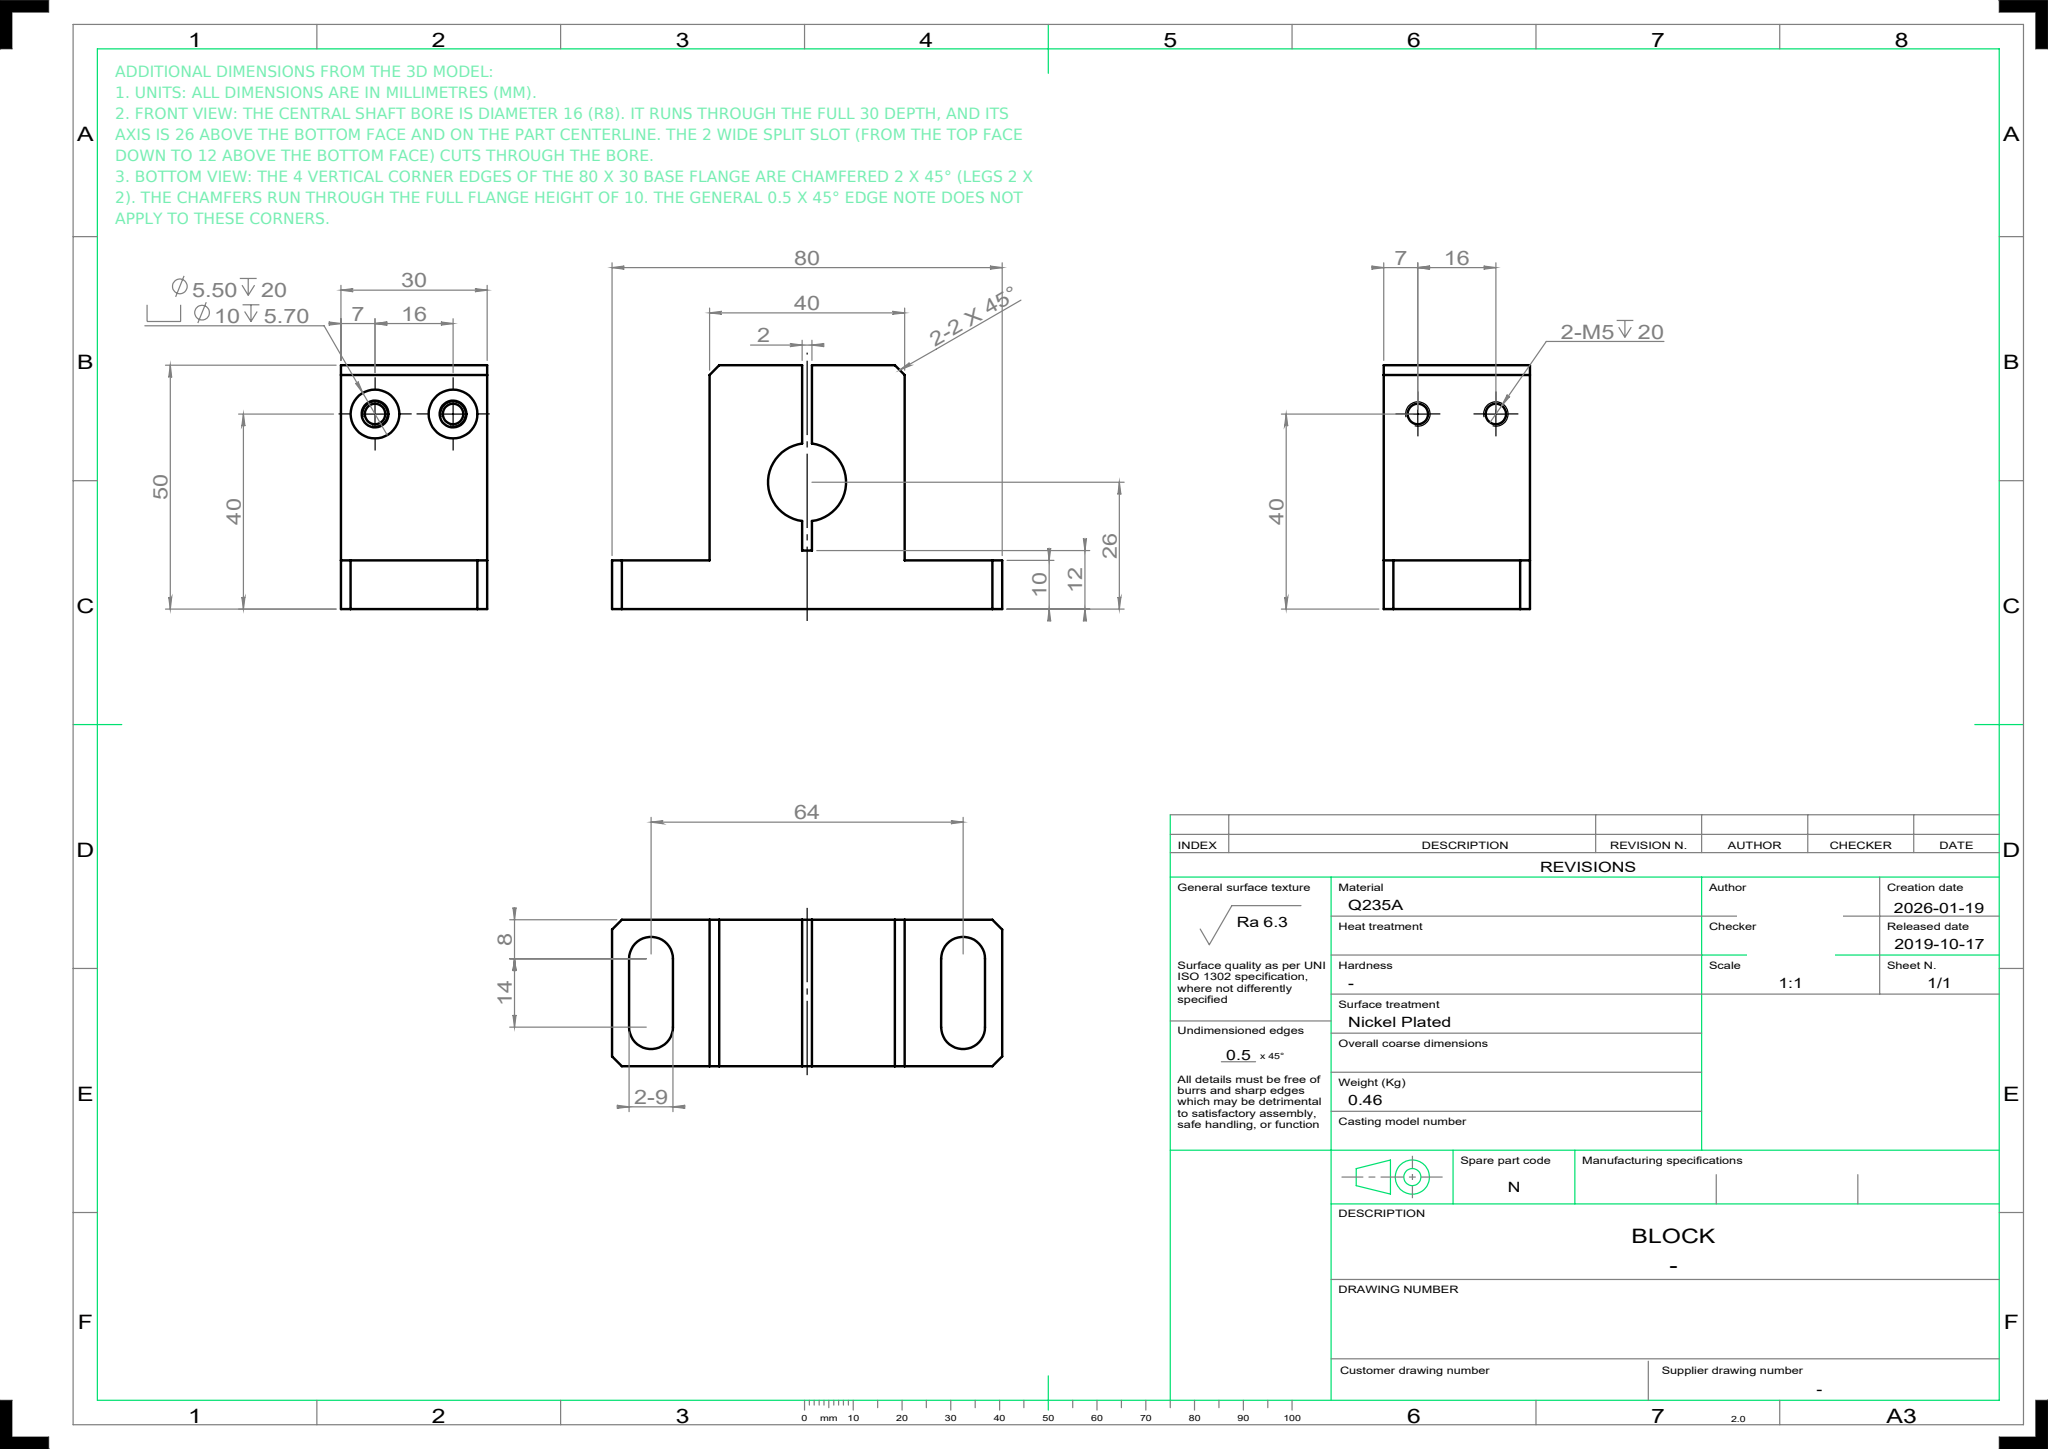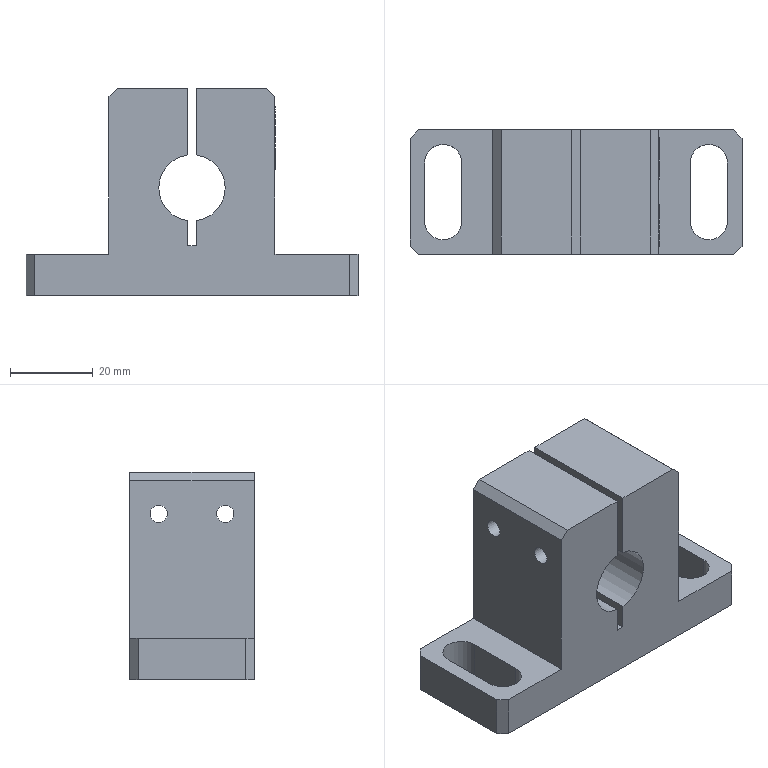Part | NX | mm | 1 solid | 40 faces | box 80 x 30 x 50 mm | volume 58599 mm3 | plane 28 | cylinder 12 | commonest cylinder face diameters 9 x4 16 x2 5.5 x2 10 x2 4.2 x2